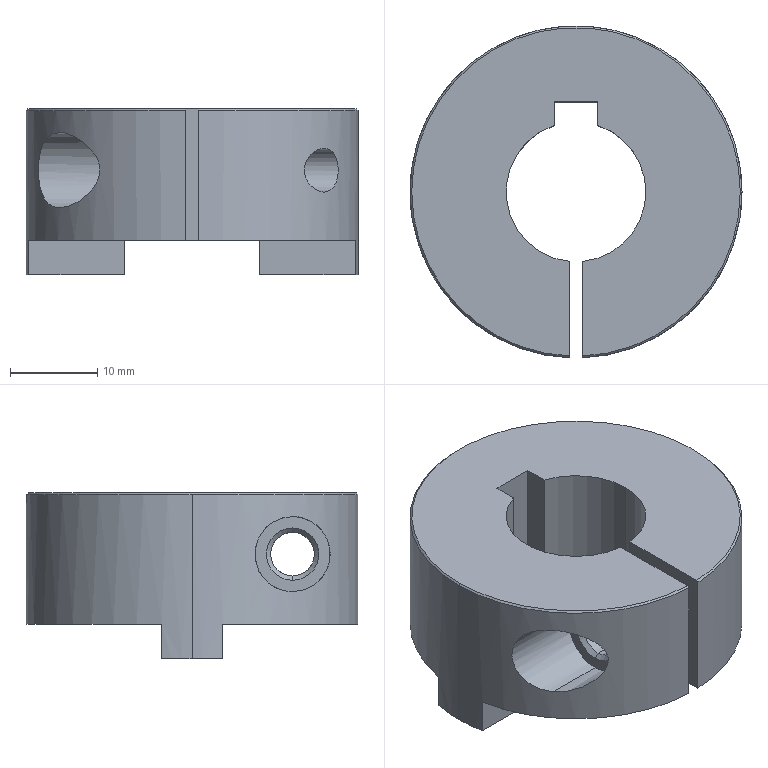Component | SolidWorks | ServoDriveMotorModule-1_MCOCGWK38_16_16-1_MCOCGXK3816-1 | 1 solid | 34 faces | box 38 x 37.99 x 19 mm | volume 13350 mm3 | cylinder 15 | plane 14 | cone 5 | commonest cylinder face diameters 5 x4 17 x3 38 x3 16 x3 8.6 x2 | material AISI 1045 Steel, cold drawn
build123d program:
from build123d import *

# Parameters (mm, degrees)
SKETCH2_W                   = 4
SKETCH2_H                   = 8.5
SKETCH3_W                   = 1.5
SKETCH3_H                   = 19
CUT_EXTRUDE1_DEPTH          = 15
SKETCH6_W                   = 40
SKETCH6_H                   = 39
SKETCH6_W_2                 = 38
SKETCH6_H_2                 = 7
CUT_EXTRUDE2_DEPTH          = 4
SKETCH7_W                   = 5
SKETCH7_H                   = 10.3
CUT_EXTRUDE3_DEPTH          = 19
M5_TAPBORE_SKETCH_R         = 2.5
M5_TAPBORE_LINETOLINE_DEPTH = 3.5
M5_HEADSEAT_EDGEBREAK_SIZE  = 0.5


with BuildPart() as part:
    # Sketch1 → Revolve1 (revolve)
    with BuildSketch(Plane.XY, mode=Mode.PRIVATE) as revolve1_sk:
        Polygon((0, 18.8), (0, 8), (19, 8), (19, 19), (0.2, 19), align=None)
    revolve(revolve1_sk.sketch.rotate(Axis((19, 0, 0), (-1, 0, 0)), 270), axis=Axis((19, 0, 0), (-1, 0, 0)))

    # Sketch2 → Cut-Revolve1 (revolve, cut)
    with BuildSketch(Plane.XY, mode=Mode.PRIVATE) as cut_revolve1_sk:
        with Locations((17, 4.25)):
            Rectangle(SKETCH2_W, SKETCH2_H)
    revolve(cut_revolve1_sk.sketch.rotate(Axis((19, 0, 0), (-1, 0, 0)), 270), axis=Axis((19, 0, 0), (-1, 0, 0)), mode=Mode.SUBTRACT)

    # Sketch3 → Cut-Extrude1 (cut)
    with BuildSketch(Plane(origin=(0, 0, 0), x_dir=(0, 0, -1), z_dir=(1, 0, 0))):
        with Locations((0, -9.5)):
            Rectangle(SKETCH3_W, SKETCH3_H)
    extrude(amount=CUT_EXTRUDE1_DEPTH, mode=Mode.SUBTRACT)

    # Sketch5 → Cut-Revolve2 (revolve, cut)
    with BuildSketch(Plane(origin=(7, 0, 0), x_dir=(0, 0, -1), z_dir=(1, 0, 0)), mode=Mode.PRIVATE) as cut_revolve2_sk:
        Polygon((-0.75, -11.5), (-0.75, -14), (-1.183, -13.567), (-2.667, -13.567), (-3.1, -14), (-3.1, -11.5), align=None)
    revolve(cut_revolve2_sk.sketch.rotate(Axis((7, -11.5, 3.1), (0, 0, -1)), 90), axis=Axis((7, -11.5, 3.1), (0, 0, -1)), mode=Mode.SUBTRACT)

    # Sketch4 → Cut-Revolve3 (revolve, cut)
    with BuildSketch(Plane(origin=(7, 0, 0), x_dir=(0, 0, -1), z_dir=(1, 0, 0)), mode=Mode.PRIVATE) as cut_revolve3_sk:
        Polygon((19, -11.5), (19, -15.8), (8.4, -15.8), (8.4, -14), (-0.75, -14), (-0.75, -11.6), (-3.1, -11.6), (-3.1, -14), (-19, -14), (-19, -11.5), align=None)
    revolve(cut_revolve3_sk.sketch.rotate(Axis((7, -11.5, 19), (0, 0, -1)), 90), axis=Axis((7, -11.5, 19), (0, 0, -1)), mode=Mode.SUBTRACT)

    # Sketch6 → Cut-Extrude2 (cut)
    with BuildSketch(Plane(origin=(19, 0, 0), x_dir=(0, 0, -1), z_dir=(1, 0, 0))):
        Rectangle(SKETCH6_W, SKETCH6_H)
        Rectangle(SKETCH6_W_2, SKETCH6_H_2, mode=Mode.SUBTRACT)
    extrude(amount=-CUT_EXTRUDE2_DEPTH, mode=Mode.SUBTRACT)

    # Sketch7 → Cut-Extrude3 (cut)
    with BuildSketch(Plane(origin=(0, 0, 0), x_dir=(0, 0, -1), z_dir=(1, 0, 0))):
        with Locations((0, 5.15)):
            Rectangle(SKETCH7_W, SKETCH7_H)
    extrude(amount=CUT_EXTRUDE3_DEPTH, mode=Mode.SUBTRACT)

    # M5_TapBore_Sketch → M5_TapBore_LineToLine (cut, symmetric)
    with BuildSketch(Plane.XY):
        with Locations(Location((7, -11.5, 0), (0, 0, 180))):
            Circle(M5_TAPBORE_SKETCH_R)
    extrude(amount=M5_TAPBORE_LINETOLINE_DEPTH, both=True, mode=Mode.SUBTRACT)

    # M5_HeadSeat_EdgeBreak
    m5_headseat_edgebreak_edges = [part.edges().sort_by_distance(p)[0] for p in [
        (9.5, -11.5, -8.4),
    ]]
    chamfer(m5_headseat_edgebreak_edges, length=M5_HEADSEAT_EDGEBREAK_SIZE)


solid = part.part

# Placed as in the assembly
solid = solid.moved(Location((0, -0.0001624, 116), (0, 90, 0)))